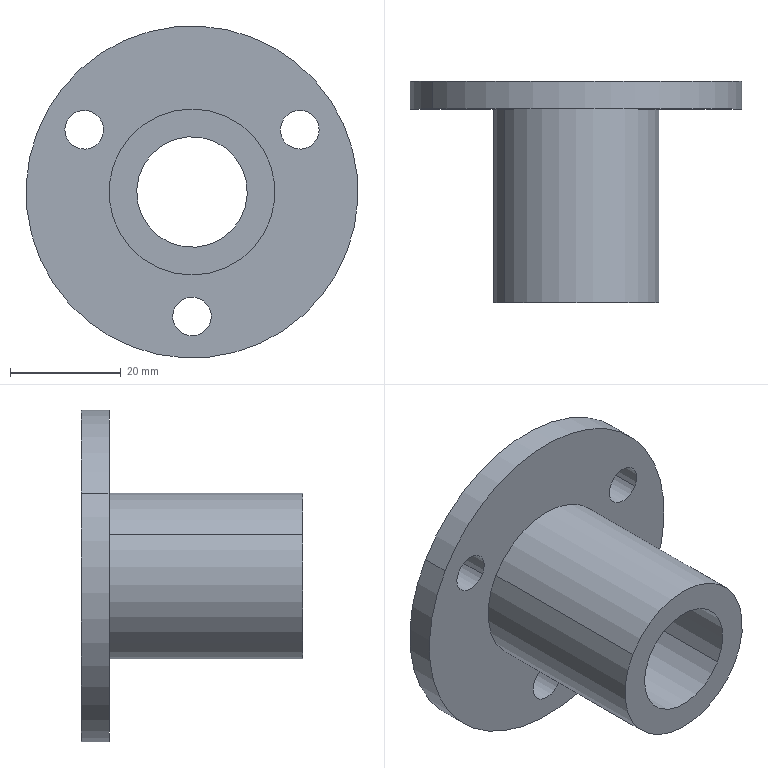Component | SolidWorks | E003CopperSleeve-1 | 1 solid | 15 faces | box 60 x 40 x 60 mm | volume 25734 mm3 | cylinder 12 | plane 3 | commonest cylinder face diameters 7 x6 60 x2 30 x2 20 x2 | material Brass
build123d program:
from build123d import *

# Parameters (mm, degrees)
SKETCH2_R          = 3.5
CUT_EXTRUDE1_DEPTH = 59.31
CIRPATTERN1_COUNT  = 3


with BuildPart() as part:
    # Sketch1 → Revolve1 (revolve)
    with BuildSketch(Plane.XY, mode=Mode.PRIVATE) as revolve1_sk:
        Polygon((10, 40), (15, 40), (15, 5), (30, 5), (30, 0), (10, 0), align=None)
    revolve(revolve1_sk.sketch.rotate(Axis((0, 0, 0), (0, 1, 0)), 90), axis=Axis((0, 0, 0), (0, 1, 0)))

    # Sketch2 → Cut-Extrude1 (cut, through all)
    with BuildSketch(Plane.XZ):
        with Locations(Location((0, 22.5, 0), (0, 0, 270))):
            Circle(SKETCH2_R)
    cut_extrude1 = extrude(amount=-CUT_EXTRUDE1_DEPTH, mode=Mode.SUBTRACT)

    # CirPattern1: Cut-Extrude1 ×3 about axis
    cirpattern1_axis = Axis((0, 0, 0), (0, 1, 0))
    for i in range(1, CIRPATTERN1_COUNT):
        add(cut_extrude1.rotate(cirpattern1_axis, i * 360 / CIRPATTERN1_COUNT), mode=Mode.SUBTRACT)


solid = part.part

# Placed as in the assembly
solid = solid.moved(Location((91, 218, 0), (180, 0, 0)))
STEP:
#1=COLOUR_RGB('',0.7922,0.8196,0.9333);
#2=FILL_AREA_STYLE_COLOUR('',#1);
#3=FILL_AREA_STYLE('',(#2));
#4=SURFACE_STYLE_FILL_AREA(#3);
#5=SURFACE_SIDE_STYLE('',(#4));
#6=SURFACE_STYLE_USAGE(.BOTH.,#5);
#7=PRESENTATION_STYLE_ASSIGNMENT((#6));
#8=CARTESIAN_POINT('',(3.702,8.386,-0.9547));
#9=VERTEX_POINT('',#8);
#10=CARTESIAN_POINT('',(3.463,8.386,-0.8169));
#11=VERTEX_POINT('',#10);
#12=CARTESIAN_POINT('',(3.583,8.386,-0.8858));
#13=DIRECTION('',(0.,-1.,0.));
#14=DIRECTION('',(-0.866,0.,0.5));
#15=AXIS2_PLACEMENT_3D('',#12,#13,#14);
#16=CIRCLE('',#15,0.1378);
#17=EDGE_CURVE('',#9,#11,#16,.T.);
#18=ORIENTED_EDGE('',*,*,#17,.T.);
#19=CARTESIAN_POINT('',(3.463,8.583,-0.8169));
#20=VERTEX_POINT('',#19);
#21=CARTESIAN_POINT('',(3.463,7.008,-0.8169));
#22=DIRECTION('',(0.,1.,0.));
#23=VECTOR('',#22,39.37);
#24=LINE('',#21,#23);
#25=EDGE_CURVE('',#11,#20,#24,.T.);
#26=ORIENTED_EDGE('',*,*,#25,.T.);
#27=CARTESIAN_POINT('',(3.702,8.583,-0.9547));
#28=VERTEX_POINT('',#27);
#29=CARTESIAN_POINT('',(3.583,8.583,-0.8858));
#30=DIRECTION('',(0.,1.,0.));
#31=DIRECTION('',(0.,0.,1.));
#32=AXIS2_PLACEMENT_3D('',#29,#30,#31);
#33=CIRCLE('',#32,0.1378);
#34=EDGE_CURVE('',#20,#28,#33,.T.);
#35=ORIENTED_EDGE('',*,*,#34,.T.);
#36=CARTESIAN_POINT('',(3.702,7.008,-0.9547));
#37=DIRECTION('',(0.,1.,0.));
#38=VECTOR('',#37,39.37);
#39=LINE('',#36,#38);
#40=EDGE_CURVE('',#9,#28,#39,.T.);
#41=ORIENTED_EDGE('',*,*,#40,.F.);
#42=EDGE_LOOP('',(#18,#26,#35,#41));
#43=FACE_OUTER_BOUND('',#42,.T.);
#44=CARTESIAN_POINT('',(3.583,7.008,-0.8858));
#45=DIRECTION('',(0.,1.,0.));
#46=DIRECTION('',(0.866,0.,-0.5));
#47=AXIS2_PLACEMENT_3D('',#44,#45,#46);
#48=CYLINDRICAL_SURFACE('',#47,0.1378);
#49=ADVANCED_FACE('',(#43),#48,.F.);
#50=CARTESIAN_POINT('',(4.469,8.386,0.374));
#51=VERTEX_POINT('',#50);
#52=CARTESIAN_POINT('',(4.23,8.386,0.5118));
#53=VERTEX_POINT('',#52);
#54=CARTESIAN_POINT('',(4.35,8.386,0.4429));
#55=DIRECTION('',(0.,-1.,0.));
#56=DIRECTION('',(-0.866,0.,0.5));
#57=AXIS2_PLACEMENT_3D('',#54,#55,#56);
#58=CIRCLE('',#57,0.1378);
#59=EDGE_CURVE('',#51,#53,#58,.T.);
#60=ORIENTED_EDGE('',*,*,#59,.T.);
#61=CARTESIAN_POINT('',(4.23,8.583,0.5118));
#62=VERTEX_POINT('',#61);
#63=CARTESIAN_POINT('',(4.23,7.008,0.5118));
#64=DIRECTION('',(0.,1.,0.));
#65=VECTOR('',#64,39.37);
#66=LINE('',#63,#65);
#67=EDGE_CURVE('',#53,#62,#66,.T.);
#68=ORIENTED_EDGE('',*,*,#67,.T.);
#69=CARTESIAN_POINT('',(4.469,8.583,0.374));
#70=VERTEX_POINT('',#69);
#71=CARTESIAN_POINT('',(4.35,8.583,0.4429));
#72=DIRECTION('',(0.,1.,0.));
#73=DIRECTION('',(-0.866,0.,-0.5));
#74=AXIS2_PLACEMENT_3D('',#71,#72,#73);
#75=CIRCLE('',#74,0.1378);
#76=EDGE_CURVE('',#62,#70,#75,.T.);
#77=ORIENTED_EDGE('',*,*,#76,.T.);
#78=CARTESIAN_POINT('',(4.469,7.008,0.374));
#79=DIRECTION('',(0.,1.,0.));
#80=VECTOR('',#79,39.37);
#81=LINE('',#78,#80);
#82=EDGE_CURVE('',#51,#70,#81,.T.);
#83=ORIENTED_EDGE('',*,*,#82,.F.);
#84=EDGE_LOOP('',(#60,#68,#77,#83));
#85=FACE_OUTER_BOUND('',#84,.T.);
#86=CARTESIAN_POINT('',(4.35,7.008,0.4429));
#87=DIRECTION('',(0.,1.,0.));
#88=DIRECTION('',(0.866,0.,-0.5));
#89=AXIS2_PLACEMENT_3D('',#86,#87,#88);
#90=CYLINDRICAL_SURFACE('',#89,0.1378);
#91=ADVANCED_FACE('',(#85),#90,.F.);
#92=CARTESIAN_POINT('',(2.935,8.386,0.374));
#93=VERTEX_POINT('',#92);
#94=CARTESIAN_POINT('',(2.696,8.386,0.5118));
#95=VERTEX_POINT('',#94);
#96=CARTESIAN_POINT('',(2.816,8.386,0.4429));
#97=DIRECTION('',(0.,-1.,0.));
#98=DIRECTION('',(-0.866,0.,0.5));
#99=AXIS2_PLACEMENT_3D('',#96,#97,#98);
#100=CIRCLE('',#99,0.1378);
#101=EDGE_CURVE('',#93,#95,#100,.T.);
#102=ORIENTED_EDGE('',*,*,#101,.T.);
#103=CARTESIAN_POINT('',(2.696,8.583,0.5118));
#104=VERTEX_POINT('',#103);
#105=CARTESIAN_POINT('',(2.696,7.008,0.5118));
#106=DIRECTION('',(0.,1.,0.));
#107=VECTOR('',#106,39.37);
#108=LINE('',#105,#107);
#109=EDGE_CURVE('',#95,#104,#108,.T.);
#110=ORIENTED_EDGE('',*,*,#109,.T.);
#111=CARTESIAN_POINT('',(2.935,8.583,0.374));
#112=VERTEX_POINT('',#111);
#113=CARTESIAN_POINT('',(2.816,8.583,0.4429));
#114=DIRECTION('',(0.,1.,0.));
#115=DIRECTION('',(0.866,0.,-0.5));
#116=AXIS2_PLACEMENT_3D('',#113,#114,#115);
#117=CIRCLE('',#116,0.1378);
#118=EDGE_CURVE('',#104,#112,#117,.T.);
#119=ORIENTED_EDGE('',*,*,#118,.T.);
#120=CARTESIAN_POINT('',(2.935,7.008,0.374));
#121=DIRECTION('',(0.,1.,0.));
#122=VECTOR('',#121,39.37);
#123=LINE('',#120,#122);
#124=EDGE_CURVE('',#93,#112,#123,.T.);
#125=ORIENTED_EDGE('',*,*,#124,.F.);
#126=EDGE_LOOP('',(#102,#110,#119,#125));
#127=FACE_OUTER_BOUND('',#126,.T.);
#128=CARTESIAN_POINT('',(2.816,7.008,0.4429));
#129=DIRECTION('',(0.,1.,0.));
#130=DIRECTION('',(0.866,0.,-0.5));
#131=AXIS2_PLACEMENT_3D('',#128,#129,#130);
#132=CYLINDRICAL_SURFACE('',#131,0.1378);
#133=ADVANCED_FACE('',(#127),#132,.F.);
#134=CARTESIAN_POINT('',(4.606,8.386,-0.5906));
#135=VERTEX_POINT('',#134);
#136=CARTESIAN_POINT('',(2.56,8.386,0.5906));
#137=VERTEX_POINT('',#136);
#138=CARTESIAN_POINT('',(3.583,8.386,-0.));
#139=DIRECTION('',(0.,1.,0.));
#140=DIRECTION('',(0.866,0.,-0.5));
#141=AXIS2_PLACEMENT_3D('',#138,#139,#140);
#142=CIRCLE('',#141,1.181);
#143=EDGE_CURVE('',#135,#137,#142,.T.);
#144=ORIENTED_EDGE('',*,*,#143,.T.);
#145=CARTESIAN_POINT('',(2.56,8.583,0.5906));
#146=VERTEX_POINT('',#145);
#147=CARTESIAN_POINT('',(2.56,8.583,0.5906));
#148=DIRECTION('',(0.,1.,0.));
#149=VECTOR('',#148,39.37);
#150=LINE('',#147,#149);
#151=EDGE_CURVE('',#137,#146,#150,.T.);
#152=ORIENTED_EDGE('',*,*,#151,.T.);
#153=CARTESIAN_POINT('',(4.606,8.583,-0.5906));
#154=VERTEX_POINT('',#153);
#155=CARTESIAN_POINT('',(3.583,8.583,-0.));
#156=DIRECTION('',(0.,1.,0.));
#157=DIRECTION('',(0.866,0.,-0.5));
#158=AXIS2_PLACEMENT_3D('',#155,#156,#157);
#159=CIRCLE('',#158,1.181);
#160=EDGE_CURVE('',#154,#146,#159,.T.);
#161=ORIENTED_EDGE('',*,*,#160,.F.);
#162=CARTESIAN_POINT('',(4.606,8.583,-0.5906));
#163=DIRECTION('',(0.,1.,0.));
#164=VECTOR('',#163,39.37);
#165=LINE('',#162,#164);
#166=EDGE_CURVE('',#135,#154,#165,.T.);
#167=ORIENTED_EDGE('',*,*,#166,.F.);
#168=EDGE_LOOP('',(#144,#152,#161,#167));
#169=FACE_OUTER_BOUND('',#168,.T.);
#170=CARTESIAN_POINT('',(3.583,8.583,-0.));
#171=DIRECTION('',(0.,1.,0.));
#172=DIRECTION('',(0.866,0.,-0.5));
#173=AXIS2_PLACEMENT_3D('',#170,#171,#172);
#174=CYLINDRICAL_SURFACE('',#173,1.181);
#175=ADVANCED_FACE('',(#169),#174,.T.);
#176=CARTESIAN_POINT('',(4.094,7.008,-0.2953));
#177=VERTEX_POINT('',#176);
#178=CARTESIAN_POINT('',(3.071,7.008,0.2953));
#179=VERTEX_POINT('',#178);
#180=CARTESIAN_POINT('',(3.583,7.008,-0.));
#181=DIRECTION('',(0.,1.,0.));
#182=DIRECTION('',(0.866,0.,-0.5));
#183=AXIS2_PLACEMENT_3D('',#180,#181,#182);
#184=CIRCLE('',#183,0.5906);
#185=EDGE_CURVE('',#177,#179,#184,.T.);
#186=ORIENTED_EDGE('',*,*,#185,.T.);
#187=CARTESIAN_POINT('',(3.071,8.386,0.2953));
#188=VERTEX_POINT('',#187);
#189=CARTESIAN_POINT('',(3.071,8.583,0.2953));
#190=DIRECTION('',(0.,1.,0.));
#191=VECTOR('',#190,39.37);
#192=LINE('',#189,#191);
#193=EDGE_CURVE('',#179,#188,#192,.T.);
#194=ORIENTED_EDGE('',*,*,#193,.T.);
#195=CARTESIAN_POINT('',(4.094,8.386,-0.2953));
#196=VERTEX_POINT('',#195);
#197=CARTESIAN_POINT('',(3.583,8.386,-0.));
#198=DIRECTION('',(0.,1.,0.));
#199=DIRECTION('',(0.866,0.,-0.5));
#200=AXIS2_PLACEMENT_3D('',#197,#198,#199);
#201=CIRCLE('',#200,0.5906);
#202=EDGE_CURVE('',#196,#188,#201,.T.);
#203=ORIENTED_EDGE('',*,*,#202,.F.);
#204=CARTESIAN_POINT('',(4.094,8.583,-0.2953));
#205=DIRECTION('',(0.,1.,0.));
#206=VECTOR('',#205,39.37);
#207=LINE('',#204,#206);
#208=EDGE_CURVE('',#177,#196,#207,.T.);
#209=ORIENTED_EDGE('',*,*,#208,.F.);
#210=EDGE_LOOP('',(#186,#194,#203,#209));
#211=FACE_OUTER_BOUND('',#210,.T.);
#212=CARTESIAN_POINT('',(3.583,8.583,-0.));
#213=DIRECTION('',(0.,1.,0.));
#214=DIRECTION('',(0.866,0.,-0.5));
#215=AXIS2_PLACEMENT_3D('',#212,#213,#214);
#216=CYLINDRICAL_SURFACE('',#215,0.5906);
#217=ADVANCED_FACE('',(#211),#216,.T.);
#218=CARTESIAN_POINT('',(3.242,7.008,0.1969));
#219=VERTEX_POINT('',#218);
#220=CARTESIAN_POINT('',(3.924,7.008,-0.1969));
#221=VERTEX_POINT('',#220);
#222=CARTESIAN_POINT('',(3.583,7.008,-0.));
#223=DIRECTION('',(0.,1.,0.));
#224=DIRECTION('',(0.866,0.,-0.5));
#225=AXIS2_PLACEMENT_3D('',#222,#223,#224);
#226=CIRCLE('',#225,0.3937);
#227=EDGE_CURVE('',#219,#221,#226,.T.);
#228=ORIENTED_EDGE('',*,*,#227,.F.);
#229=CARTESIAN_POINT('',(3.242,8.583,0.1969));
#230=VERTEX_POINT('',#229);
#231=CARTESIAN_POINT('',(3.242,8.583,0.1969));
#232=DIRECTION('',(0.,1.,0.));
#233=VECTOR('',#232,39.37);
#234=LINE('',#231,#233);
#235=EDGE_CURVE('',#219,#230,#234,.T.);
#236=ORIENTED_EDGE('',*,*,#235,.T.);
#237=CARTESIAN_POINT('',(3.924,8.583,-0.1969));
#238=VERTEX_POINT('',#237);
#239=CARTESIAN_POINT('',(3.583,8.583,-0.));
#240=DIRECTION('',(0.,1.,0.));
#241=DIRECTION('',(0.866,0.,-0.5));
#242=AXIS2_PLACEMENT_3D('',#239,#240,#241);
#243=CIRCLE('',#242,0.3937);
#244=EDGE_CURVE('',#230,#238,#243,.T.);
#245=ORIENTED_EDGE('',*,*,#244,.T.);
#246=CARTESIAN_POINT('',(3.924,8.583,-0.1969));
#247=DIRECTION('',(0.,1.,0.));
#248=VECTOR('',#247,39.37);
#249=LINE('',#246,#248);
#250=EDGE_CURVE('',#221,#238,#249,.T.);
#251=ORIENTED_EDGE('',*,*,#250,.F.);
#252=EDGE_LOOP('',(#228,#236,#245,#251));
#253=FACE_OUTER_BOUND('',#252,.T.);
#254=CARTESIAN_POINT('',(3.583,8.583,-0.));
#255=DIRECTION('',(0.,1.,0.));
#256=DIRECTION('',(0.866,0.,-0.5));
#257=AXIS2_PLACEMENT_3D('',#254,#255,#256);
#258=CYLINDRICAL_SURFACE('',#257,0.3937);
#259=ADVANCED_FACE('',(#253),#258,.F.);
#260=ORIENTED_EDGE('',*,*,#235,.F.);
#261=CARTESIAN_POINT('',(3.583,7.008,-0.));
#262=DIRECTION('',(0.,1.,0.));
#263=DIRECTION('',(0.866,0.,-0.5));
#264=AXIS2_PLACEMENT_3D('',#261,#262,#263);
#265=CIRCLE('',#264,0.3937);
#266=EDGE_CURVE('',#221,#219,#265,.T.);
#267=ORIENTED_EDGE('',*,*,#266,.F.);
#268=ORIENTED_EDGE('',*,*,#250,.T.);
#269=CARTESIAN_POINT('',(3.583,8.583,-0.));
#270=DIRECTION('',(0.,1.,0.));
#271=DIRECTION('',(0.866,0.,-0.5));
#272=AXIS2_PLACEMENT_3D('',#269,#270,#271);
#273=CIRCLE('',#272,0.3937);
#274=EDGE_CURVE('',#238,#230,#273,.T.);
#275=ORIENTED_EDGE('',*,*,#274,.T.);
#276=EDGE_LOOP('',(#260,#267,#268,#275));
#277=FACE_OUTER_BOUND('',#276,.T.);
#278=CARTESIAN_POINT('',(3.583,8.583,-0.));
#279=DIRECTION('',(0.,1.,0.));
#280=DIRECTION('',(0.866,0.,-0.5));
#281=AXIS2_PLACEMENT_3D('',#278,#279,#280);
#282=CYLINDRICAL_SURFACE('',#281,0.3937);
#283=ADVANCED_FACE('',(#277),#282,.F.);
#284=ORIENTED_EDGE('',*,*,#266,.T.);
#285=ORIENTED_EDGE('',*,*,#227,.T.);
#286=EDGE_LOOP('',(#284,#285));
#287=FACE_BOUND('',#286,.T.);
#288=ORIENTED_EDGE('',*,*,#185,.F.);
#289=CARTESIAN_POINT('',(3.583,7.008,-0.));
#290=DIRECTION('',(0.,1.,0.));
#291=DIRECTION('',(0.866,0.,-0.5));
#292=AXIS2_PLACEMENT_3D('',#289,#290,#291);
#293=CIRCLE('',#292,0.5906);
#294=EDGE_CURVE('',#179,#177,#293,.T.);
#295=ORIENTED_EDGE('',*,*,#294,.F.);
#296=EDGE_LOOP('',(#288,#295));
#297=FACE_OUTER_BOUND('',#296,.T.);
#298=CARTESIAN_POINT('',(3.386,7.008,-0.341));
#299=DIRECTION('',(0.,-1.,0.));
#300=DIRECTION('',(-0.866,0.,0.5));
#301=AXIS2_PLACEMENT_3D('',#298,#299,#300);
#302=PLANE('',#301);
#303=ADVANCED_FACE('',(#287,#297),#302,.T.);
#304=ORIENTED_EDGE('',*,*,#193,.F.);
#305=ORIENTED_EDGE('',*,*,#294,.T.);
#306=ORIENTED_EDGE('',*,*,#208,.T.);
#307=CARTESIAN_POINT('',(3.583,8.386,-0.));
#308=DIRECTION('',(0.,1.,0.));
#309=DIRECTION('',(0.866,0.,-0.5));
#310=AXIS2_PLACEMENT_3D('',#307,#308,#309);
#311=CIRCLE('',#310,0.5906);
#312=EDGE_CURVE('',#188,#196,#311,.T.);
#313=ORIENTED_EDGE('',*,*,#312,.F.);
#314=EDGE_LOOP('',(#304,#305,#306,#313));
#315=FACE_OUTER_BOUND('',#314,.T.);
#316=CARTESIAN_POINT('',(3.583,8.583,-0.));
#317=DIRECTION('',(0.,1.,0.));
#318=DIRECTION('',(0.866,0.,-0.5));
#319=AXIS2_PLACEMENT_3D('',#316,#317,#318);
#320=CYLINDRICAL_SURFACE('',#319,0.5906);
#321=ADVANCED_FACE('',(#315),#320,.T.);
#322=ORIENTED_EDGE('',*,*,#17,.F.);
#323=CARTESIAN_POINT('',(3.583,8.386,-0.8858));
#324=DIRECTION('',(0.,-1.,0.));
#325=DIRECTION('',(-0.866,0.,0.5));
#326=AXIS2_PLACEMENT_3D('',#323,#324,#325);
#327=CIRCLE('',#326,0.1378);
#328=EDGE_CURVE('',#11,#9,#327,.T.);
#329=ORIENTED_EDGE('',*,*,#328,.F.);
#330=EDGE_LOOP('',(#322,#329));
#331=FACE_BOUND('',#330,.T.);
#332=ORIENTED_EDGE('',*,*,#59,.F.);
#333=CARTESIAN_POINT('',(4.35,8.386,0.4429));
#334=DIRECTION('',(0.,-1.,0.));
#335=DIRECTION('',(-0.866,0.,0.5));
#336=AXIS2_PLACEMENT_3D('',#333,#334,#335);
#337=CIRCLE('',#336,0.1378);
#338=EDGE_CURVE('',#53,#51,#337,.T.);
#339=ORIENTED_EDGE('',*,*,#338,.F.);
#340=EDGE_LOOP('',(#332,#339));
#341=FACE_BOUND('',#340,.T.);
#342=ORIENTED_EDGE('',*,*,#101,.F.);
#343=CARTESIAN_POINT('',(2.816,8.386,0.4429));
#344=DIRECTION('',(0.,-1.,0.));
#345=DIRECTION('',(-0.866,0.,0.5));
#346=AXIS2_PLACEMENT_3D('',#343,#344,#345);
#347=CIRCLE('',#346,0.1378);
#348=EDGE_CURVE('',#95,#93,#347,.T.);
#349=ORIENTED_EDGE('',*,*,#348,.F.);
#350=EDGE_LOOP('',(#342,#349));
#351=FACE_BOUND('',#350,.T.);
#352=ORIENTED_EDGE('',*,*,#202,.T.);
#353=ORIENTED_EDGE('',*,*,#312,.T.);
#354=EDGE_LOOP('',(#352,#353));
#355=FACE_BOUND('',#354,.T.);
#356=ORIENTED_EDGE('',*,*,#143,.F.);
#357=CARTESIAN_POINT('',(3.583,8.386,-0.));
#358=DIRECTION('',(0.,1.,0.));
#359=DIRECTION('',(0.866,0.,-0.5));
#360=AXIS2_PLACEMENT_3D('',#357,#358,#359);
#361=CIRCLE('',#360,1.181);
#362=EDGE_CURVE('',#137,#135,#361,.T.);
#363=ORIENTED_EDGE('',*,*,#362,.F.);
#364=EDGE_LOOP('',(#356,#363));
#365=FACE_OUTER_BOUND('',#364,.T.);
#366=CARTESIAN_POINT('',(3.287,8.386,-0.5114));
#367=DIRECTION('',(0.,-1.,0.));
#368=DIRECTION('',(-0.866,0.,0.5));
#369=AXIS2_PLACEMENT_3D('',#366,#367,#368);
#370=PLANE('',#369);
#371=ADVANCED_FACE('',(#331,#341,#351,#355,#365),#370,.T.);
#372=ORIENTED_EDGE('',*,*,#151,.F.);
#373=ORIENTED_EDGE('',*,*,#362,.T.);
#374=ORIENTED_EDGE('',*,*,#166,.T.);
#375=CARTESIAN_POINT('',(3.583,8.583,-0.));
#376=DIRECTION('',(0.,1.,0.));
#377=DIRECTION('',(0.866,0.,-0.5));
#378=AXIS2_PLACEMENT_3D('',#375,#376,#377);
#379=CIRCLE('',#378,1.181);
#380=EDGE_CURVE('',#146,#154,#379,.T.);
#381=ORIENTED_EDGE('',*,*,#380,.F.);
#382=EDGE_LOOP('',(#372,#373,#374,#381));
#383=FACE_OUTER_BOUND('',#382,.T.);
#384=CARTESIAN_POINT('',(3.583,8.583,-0.));
#385=DIRECTION('',(0.,1.,0.));
#386=DIRECTION('',(0.866,0.,-0.5));
#387=AXIS2_PLACEMENT_3D('',#384,#385,#386);
#388=CYLINDRICAL_SURFACE('',#387,1.181);
#389=ADVANCED_FACE('',(#383),#388,.T.);
#390=CARTESIAN_POINT('',(3.583,8.583,-0.8858));
#391=DIRECTION('',(0.,1.,0.));
#392=DIRECTION('',(0.,0.,1.));
#393=AXIS2_PLACEMENT_3D('',#390,#391,#392);
#394=CIRCLE('',#393,0.1378);
#395=EDGE_CURVE('',#28,#20,#394,.T.);
#396=ORIENTED_EDGE('',*,*,#395,.F.);
#397=ORIENTED_EDGE('',*,*,#34,.F.);
#398=EDGE_LOOP('',(#396,#397));
#399=FACE_BOUND('',#398,.T.);
#400=CARTESIAN_POINT('',(4.35,8.583,0.4429));
#401=DIRECTION('',(0.,1.,0.));
#402=DIRECTION('',(-0.866,0.,-0.5));
#403=AXIS2_PLACEMENT_3D('',#400,#401,#402);
#404=CIRCLE('',#403,0.1378);
#405=EDGE_CURVE('',#70,#62,#404,.T.);
#406=ORIENTED_EDGE('',*,*,#405,.F.);
#407=ORIENTED_EDGE('',*,*,#76,.F.);
#408=EDGE_LOOP('',(#406,#407));
#409=FACE_BOUND('',#408,.T.);
#410=CARTESIAN_POINT('',(2.816,8.583,0.4429));
#411=DIRECTION('',(0.,1.,0.));
#412=DIRECTION('',(0.866,0.,-0.5));
#413=AXIS2_PLACEMENT_3D('',#410,#411,#412);
#414=CIRCLE('',#413,0.1378);
#415=EDGE_CURVE('',#112,#104,#414,.T.);
#416=ORIENTED_EDGE('',*,*,#415,.F.);
#417=ORIENTED_EDGE('',*,*,#118,.F.);
#418=EDGE_LOOP('',(#416,#417));
#419=FACE_BOUND('',#418,.T.);
#420=ORIENTED_EDGE('',*,*,#160,.T.);
#421=ORIENTED_EDGE('',*,*,#380,.T.);
#422=EDGE_LOOP('',(#420,#421));
#423=FACE_OUTER_BOUND('',#422,.T.);
#424=ORIENTED_EDGE('',*,*,#274,.F.);
#425=ORIENTED_EDGE('',*,*,#244,.F.);
#426=EDGE_LOOP('',(#424,#425));
#427=FACE_BOUND('',#426,.T.);
#428=CARTESIAN_POINT('',(2.992,8.583,-1.023));
#429=DIRECTION('',(0.,1.,0.));
#430=DIRECTION('',(0.866,0.,-0.5));
#431=AXIS2_PLACEMENT_3D('',#428,#429,#430);
#432=PLANE('',#431);
#433=ADVANCED_FACE('',(#399,#409,#419,#423,#427),#432,.T.);
#434=ORIENTED_EDGE('',*,*,#109,.F.);
#435=ORIENTED_EDGE('',*,*,#348,.T.);
#436=ORIENTED_EDGE('',*,*,#124,.T.);
#437=ORIENTED_EDGE('',*,*,#415,.T.);
#438=EDGE_LOOP('',(#434,#435,#436,#437));
#439=FACE_OUTER_BOUND('',#438,.T.);
#440=CARTESIAN_POINT('',(2.816,7.008,0.4429));
#441=DIRECTION('',(0.,1.,0.));
#442=DIRECTION('',(0.866,0.,-0.5));
#443=AXIS2_PLACEMENT_3D('',#440,#441,#442);
#444=CYLINDRICAL_SURFACE('',#443,0.1378);
#445=ADVANCED_FACE('',(#439),#444,.F.);
#446=ORIENTED_EDGE('',*,*,#67,.F.);
#447=ORIENTED_EDGE('',*,*,#338,.T.);
#448=ORIENTED_EDGE('',*,*,#82,.T.);
#449=ORIENTED_EDGE('',*,*,#405,.T.);
#450=EDGE_LOOP('',(#446,#447,#448,#449));
#451=FACE_OUTER_BOUND('',#450,.T.);
#452=CARTESIAN_POINT('',(4.35,7.008,0.4429));
#453=DIRECTION('',(0.,1.,0.));
#454=DIRECTION('',(0.866,0.,-0.5));
#455=AXIS2_PLACEMENT_3D('',#452,#453,#454);
#456=CYLINDRICAL_SURFACE('',#455,0.1378);
#457=ADVANCED_FACE('',(#451),#456,.F.);
#458=ORIENTED_EDGE('',*,*,#25,.F.);
#459=ORIENTED_EDGE('',*,*,#328,.T.);
#460=ORIENTED_EDGE('',*,*,#40,.T.);
#461=ORIENTED_EDGE('',*,*,#395,.T.);
#462=EDGE_LOOP('',(#458,#459,#460,#461));
#463=FACE_OUTER_BOUND('',#462,.T.);
#464=CARTESIAN_POINT('',(3.583,7.008,-0.8858));
#465=DIRECTION('',(0.,1.,0.));
#466=DIRECTION('',(0.866,0.,-0.5));
#467=AXIS2_PLACEMENT_3D('',#464,#465,#466);
#468=CYLINDRICAL_SURFACE('',#467,0.1378);
#469=ADVANCED_FACE('',(#463),#468,.F.);
#470=CLOSED_SHELL('',(#49,#91,#133,#175,#217,#259,#283,#303,#321,#371,#389,#433,#445,#457,#469));
#471=MANIFOLD_SOLID_BREP('',#470);
#472=STYLED_ITEM('',(#7),#471);
#473=PRESENTATION_LAYER_ASSIGNMENT('','',(#472));
#474=CARTESIAN_POINT('',(0.,0.,0.));
#475=DIRECTION('',(0.,0.,1.));
#476=DIRECTION('',(1.,0.,0.));
#477=AXIS2_PLACEMENT_3D('',#474,#475,#476);
#478=(LENGTH_UNIT()NAMED_UNIT(*)SI_UNIT($,.METRE.));
#479=LENGTH_MEASURE_WITH_UNIT(LENGTH_MEASURE(0.0254),#478);
#480=DIMENSIONAL_EXPONENTS(1.,0.,0.,0.,0.,0.,0.);
#481=(CONVERSION_BASED_UNIT('',#479)LENGTH_UNIT()NAMED_UNIT(#480));
#482=UNCERTAINTY_MEASURE_WITH_UNIT(LENGTH_MEASURE(0.00001),#481,'','');
#483=(NAMED_UNIT(*)PLANE_ANGLE_UNIT()SI_UNIT($,.RADIAN.));
#484=(NAMED_UNIT(*)SI_UNIT($,.STERADIAN.)SOLID_ANGLE_UNIT());
#485=(GEOMETRIC_REPRESENTATION_CONTEXT(3)GLOBAL_UNCERTAINTY_ASSIGNED_CONTEXT((#482))GLOBAL_UNIT_ASSIGNED_CONTEXT((#481,#483,#484))REPRESENTATION_CONTEXT('',''));
#486=ADVANCED_BREP_SHAPE_REPRESENTATION('',(#471,#477),#485);
#487=(LENGTH_UNIT()NAMED_UNIT(*)SI_UNIT($,.METRE.));
#488=LENGTH_MEASURE_WITH_UNIT(LENGTH_MEASURE(0.0254),#487);
#489=DIMENSIONAL_EXPONENTS(1.,0.,0.,0.,0.,0.,0.);
#490=(CONVERSION_BASED_UNIT('',#488)LENGTH_UNIT()NAMED_UNIT(#489));
#491=UNCERTAINTY_MEASURE_WITH_UNIT(LENGTH_MEASURE(0.00001),#490,'','');
#492=(NAMED_UNIT(*)PLANE_ANGLE_UNIT()SI_UNIT($,.RADIAN.));
#493=(NAMED_UNIT(*)SI_UNIT($,.STERADIAN.)SOLID_ANGLE_UNIT());
#494=(GEOMETRIC_REPRESENTATION_CONTEXT(3)GLOBAL_UNCERTAINTY_ASSIGNED_CONTEXT((#491))GLOBAL_UNIT_ASSIGNED_CONTEXT((#490,#492,#493))REPRESENTATION_CONTEXT('',''));
#495=MECHANICAL_DESIGN_GEOMETRIC_PRESENTATION_REPRESENTATION('',(#472),#494);